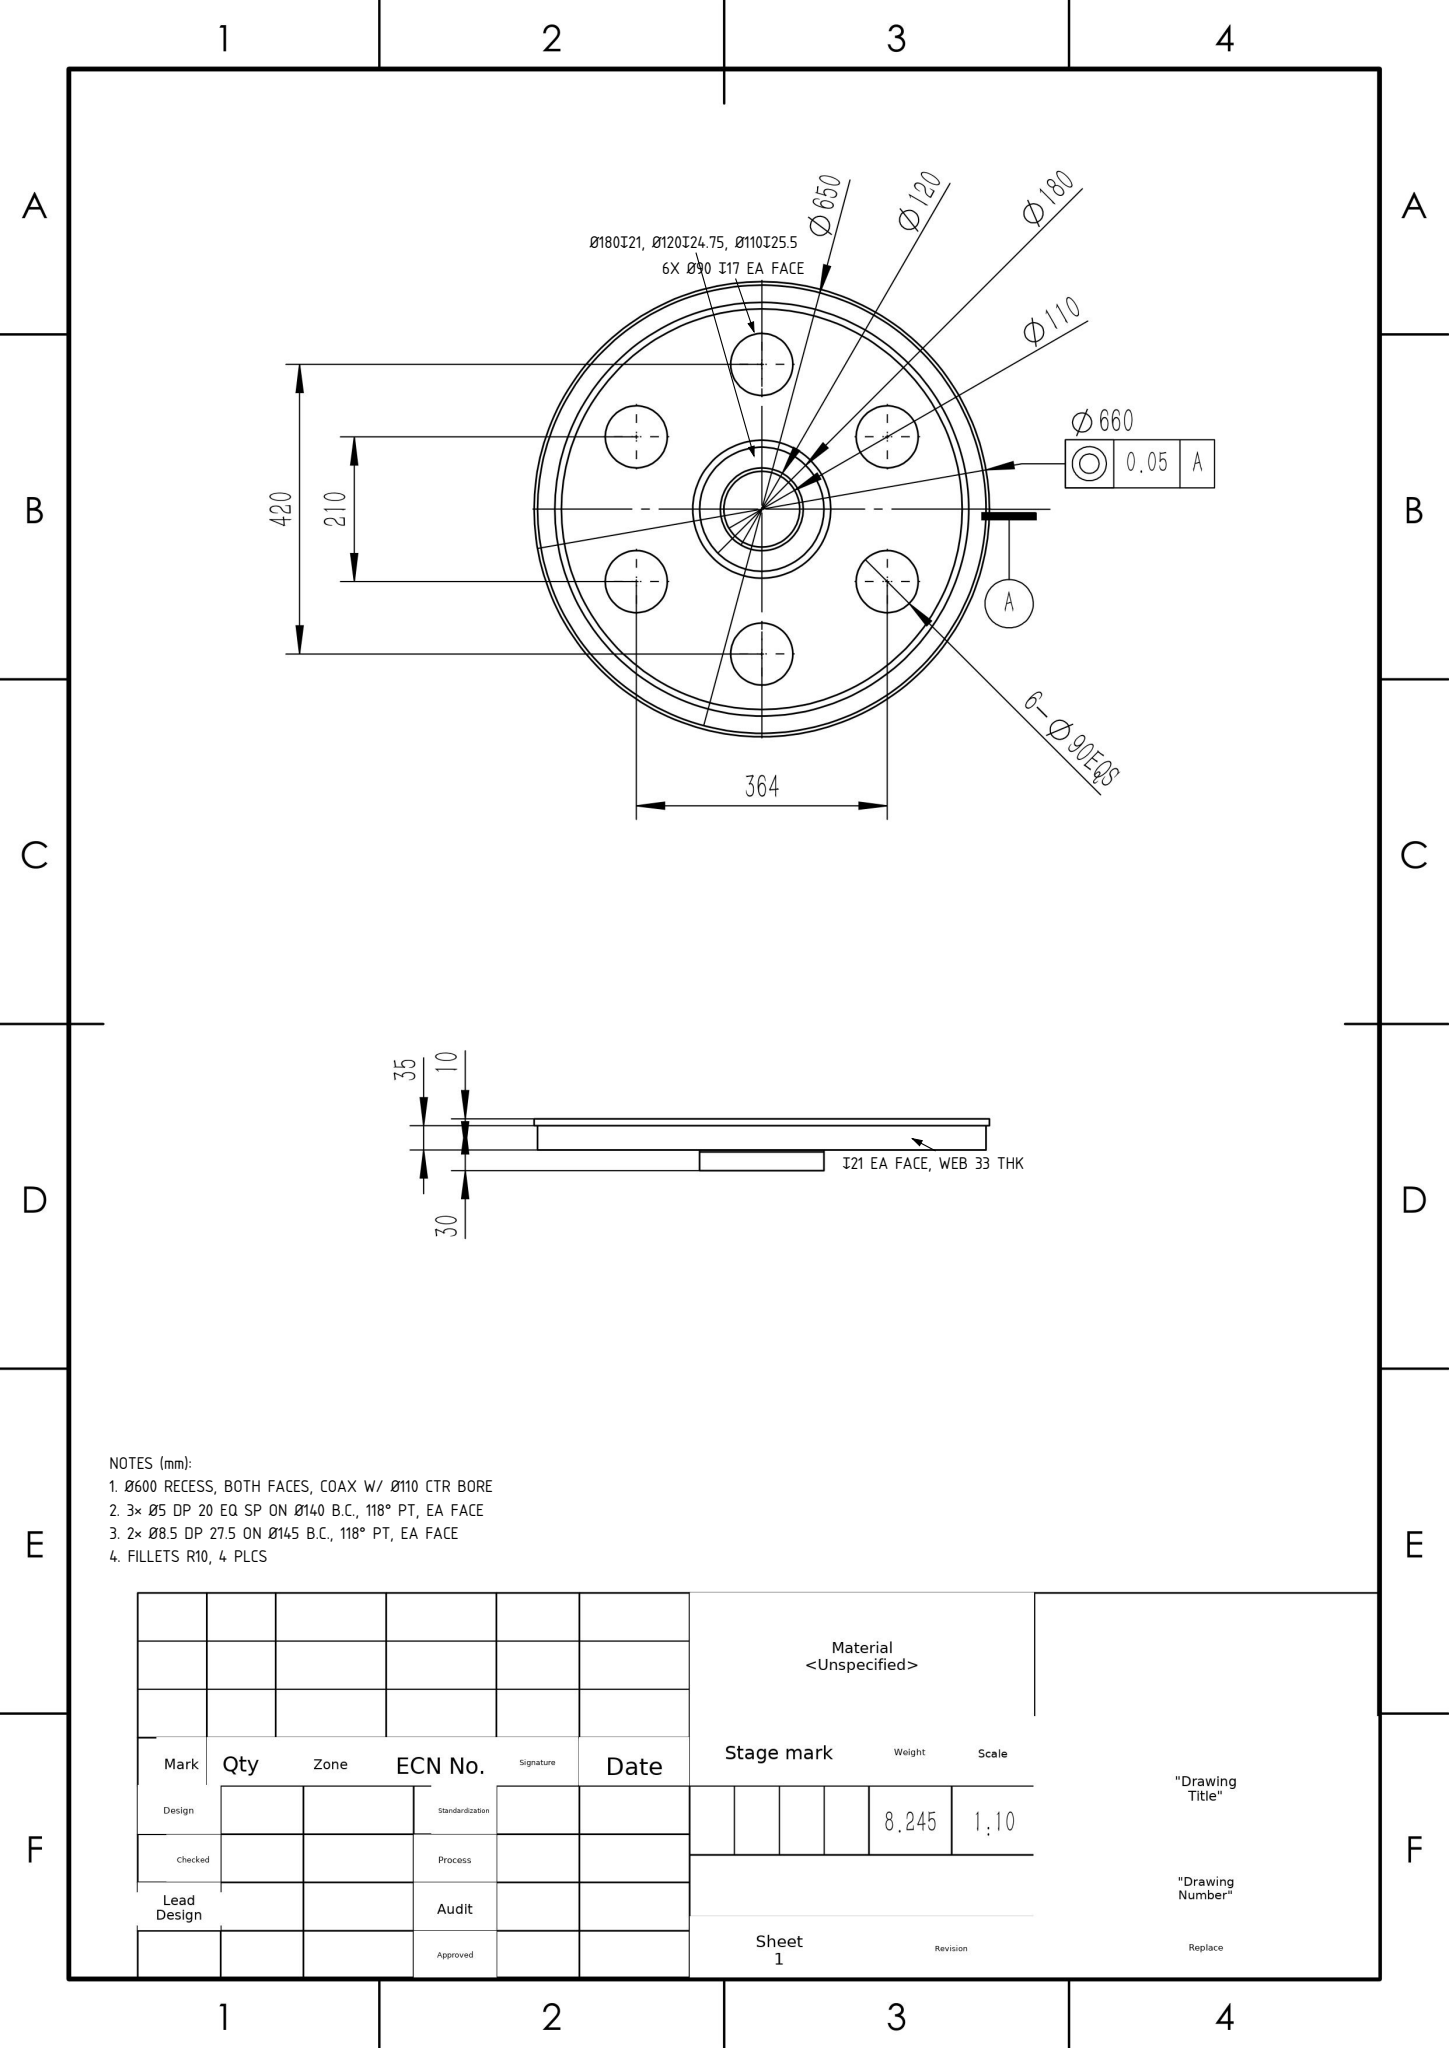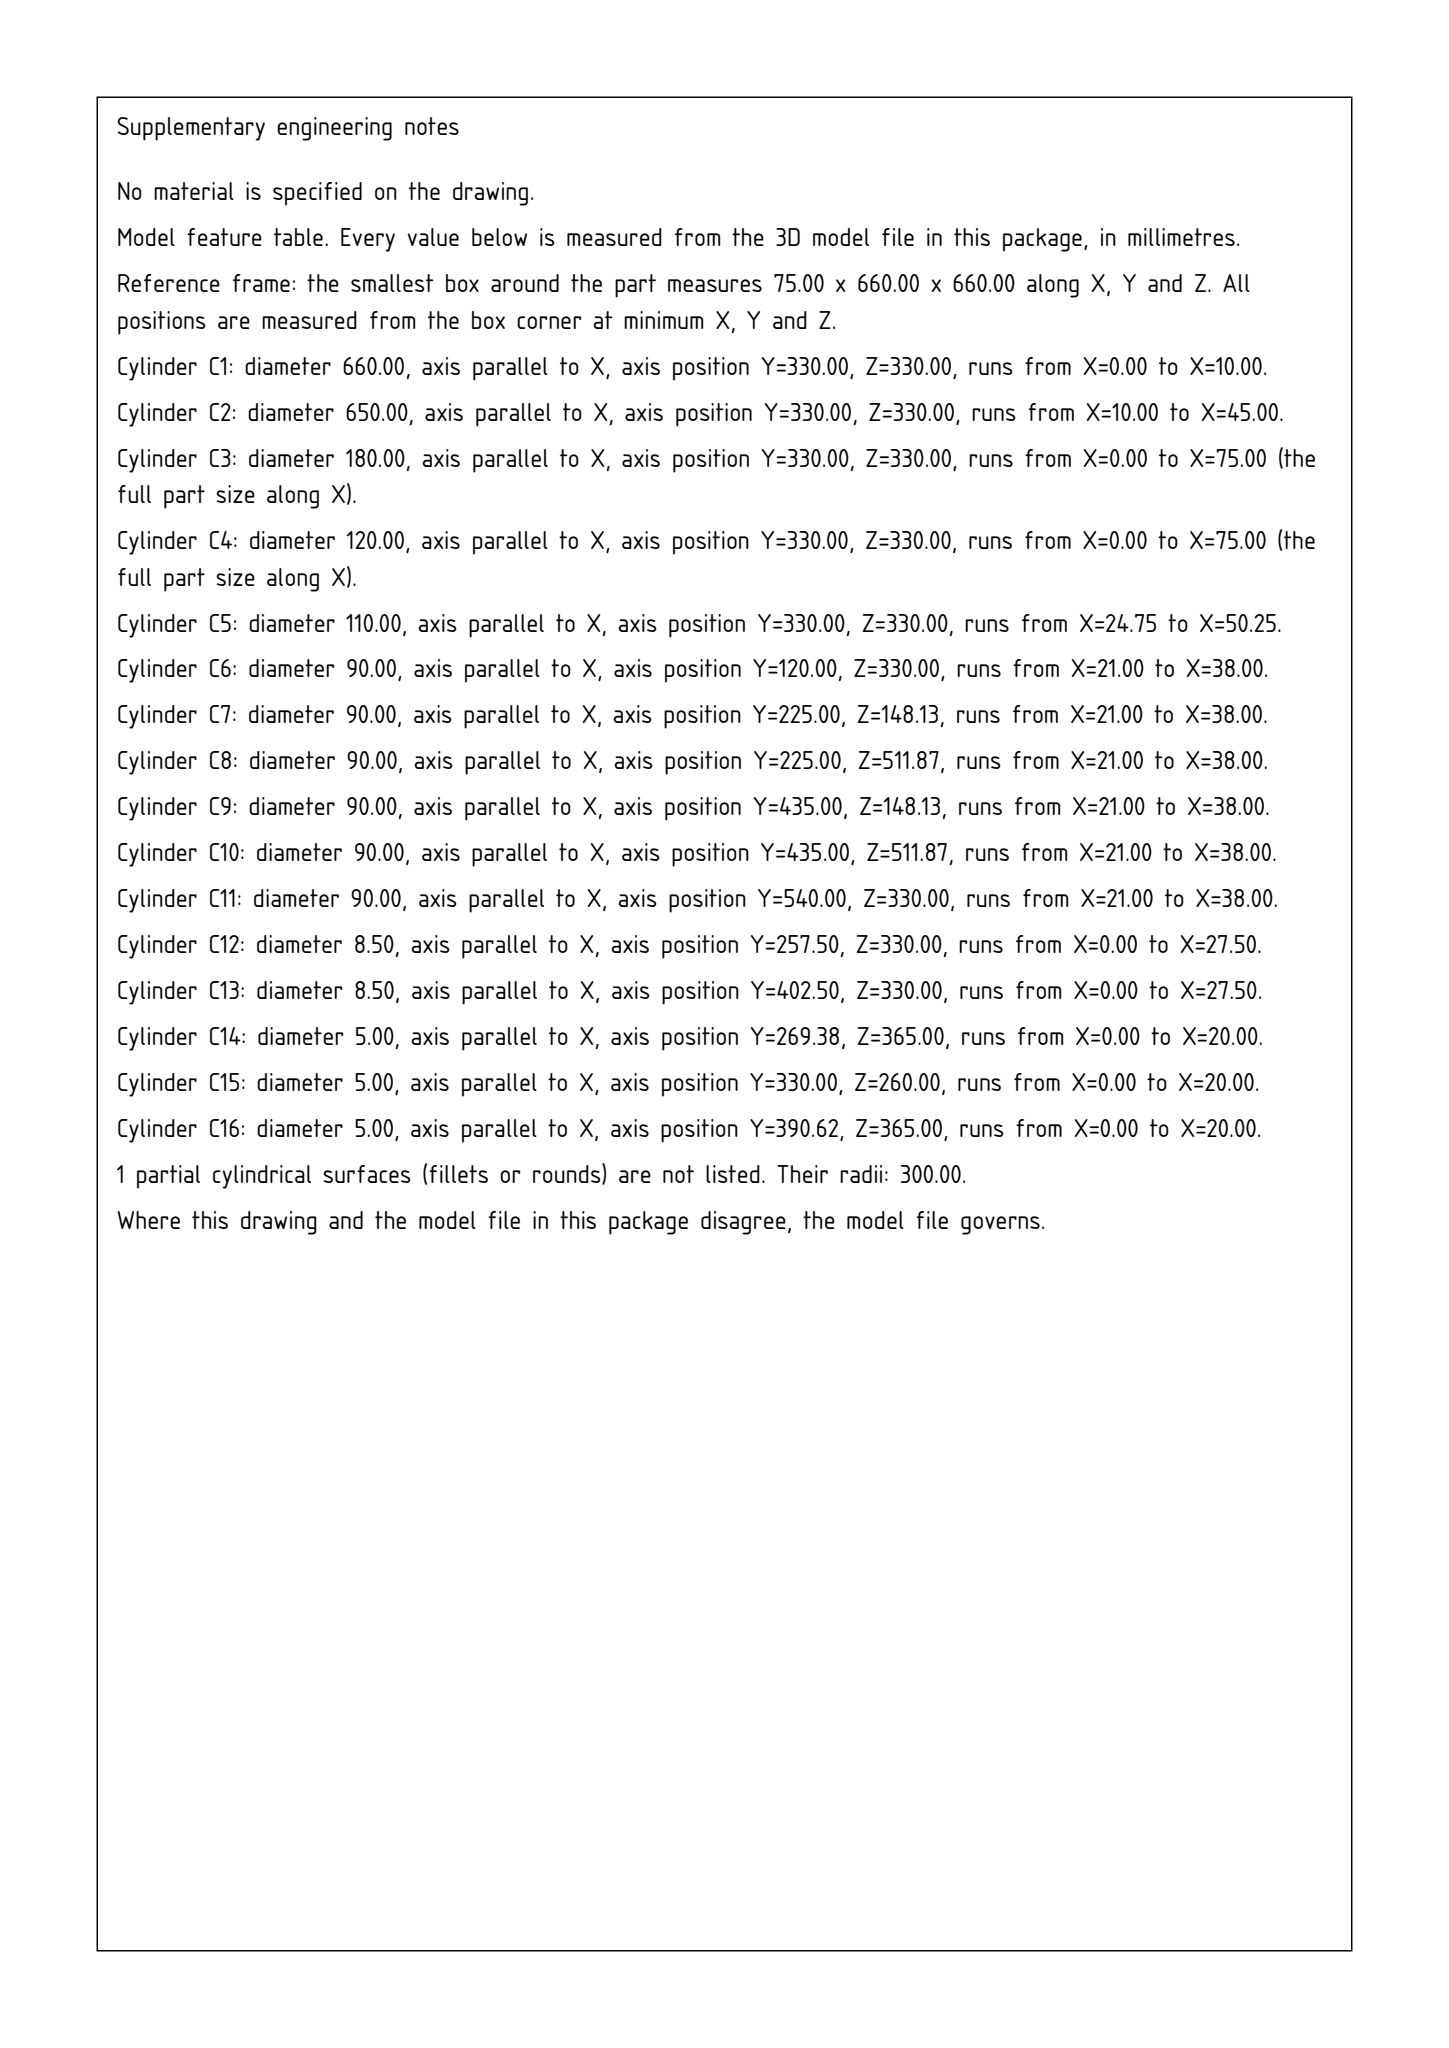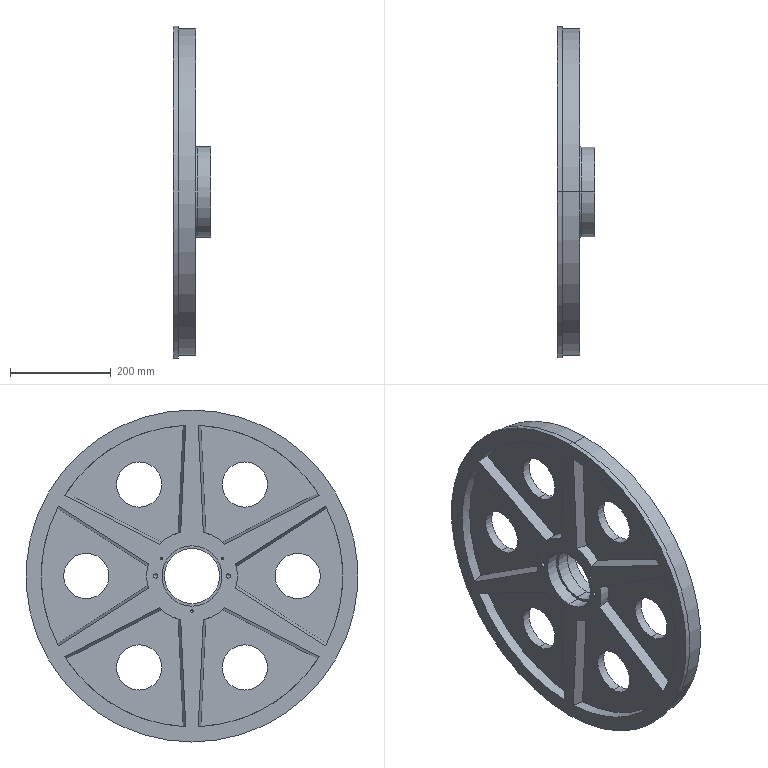Part | SolidWorks | mm | 1 solid | 97 faces | box 75 x 660 x 660 mm | volume 8244965 mm3 | cylinder 46 | spline 24 | plane 13 | cone 10 | torus 4 | commonest cylinder face diameters 90 x12 180 x8 5 x6 600 x6 8.5 x4 120 x4 110 x2 650 x2
Drawing notes:
Ø600 RECESS, BOTH FACES, COAX W/ Ø110 CTR BORE | from the solid: cyl dia 600 axis x at (y330,z330), len 21, present both faces
Ø600 RECESS DP 21 EA FACE; WEB 33 THK | from the solid: 600 dia len 21; planes x=21 & x=54 (75-21); 75-2x21=33
3× Ø5 DP 20 EQ SP ON Ø140 B.C., 118° PT, EA FACE | from the solid: Ø5 x-axis holes at (269.38,365),(330,260),(390.62,365); r=70 from ctr (330,330); len 20; cone 118°
2× Ø8.5 DP 27.5 ON Ø145 B.C., 118° PT, EA FACE | from the solid: Ø8.5 holes at (257.5,330)&(402.5,330), ±72.5 from ctr; len 27.5; cone 118°
FILLETS R10, 4 PLCS | from the solid: fillet_radii [10.0, 4]
6X Ø90 DP 17 EQ SP EA FACE (12 TOTAL) | from the solid: Six Ø90 x 17 deep cyls at Y/Z 120/330, 225/148.13, 225/511.87, 435/148.13, 435/511.87, 540/330, each count 2 (one per face, X=0 and X=75)
CTR BORE Ø180 DP 21, Ø120 DP 24.75, Ø110 DP 25.5 - EA FACE | from the solid: Coaxial cyls at Y330/Z330: Ø180 L21, Ø120 L24.75, Ø110 L25.5 blind from both X=0 and X=75 faces; planes at X=21, 24.75, 50.25